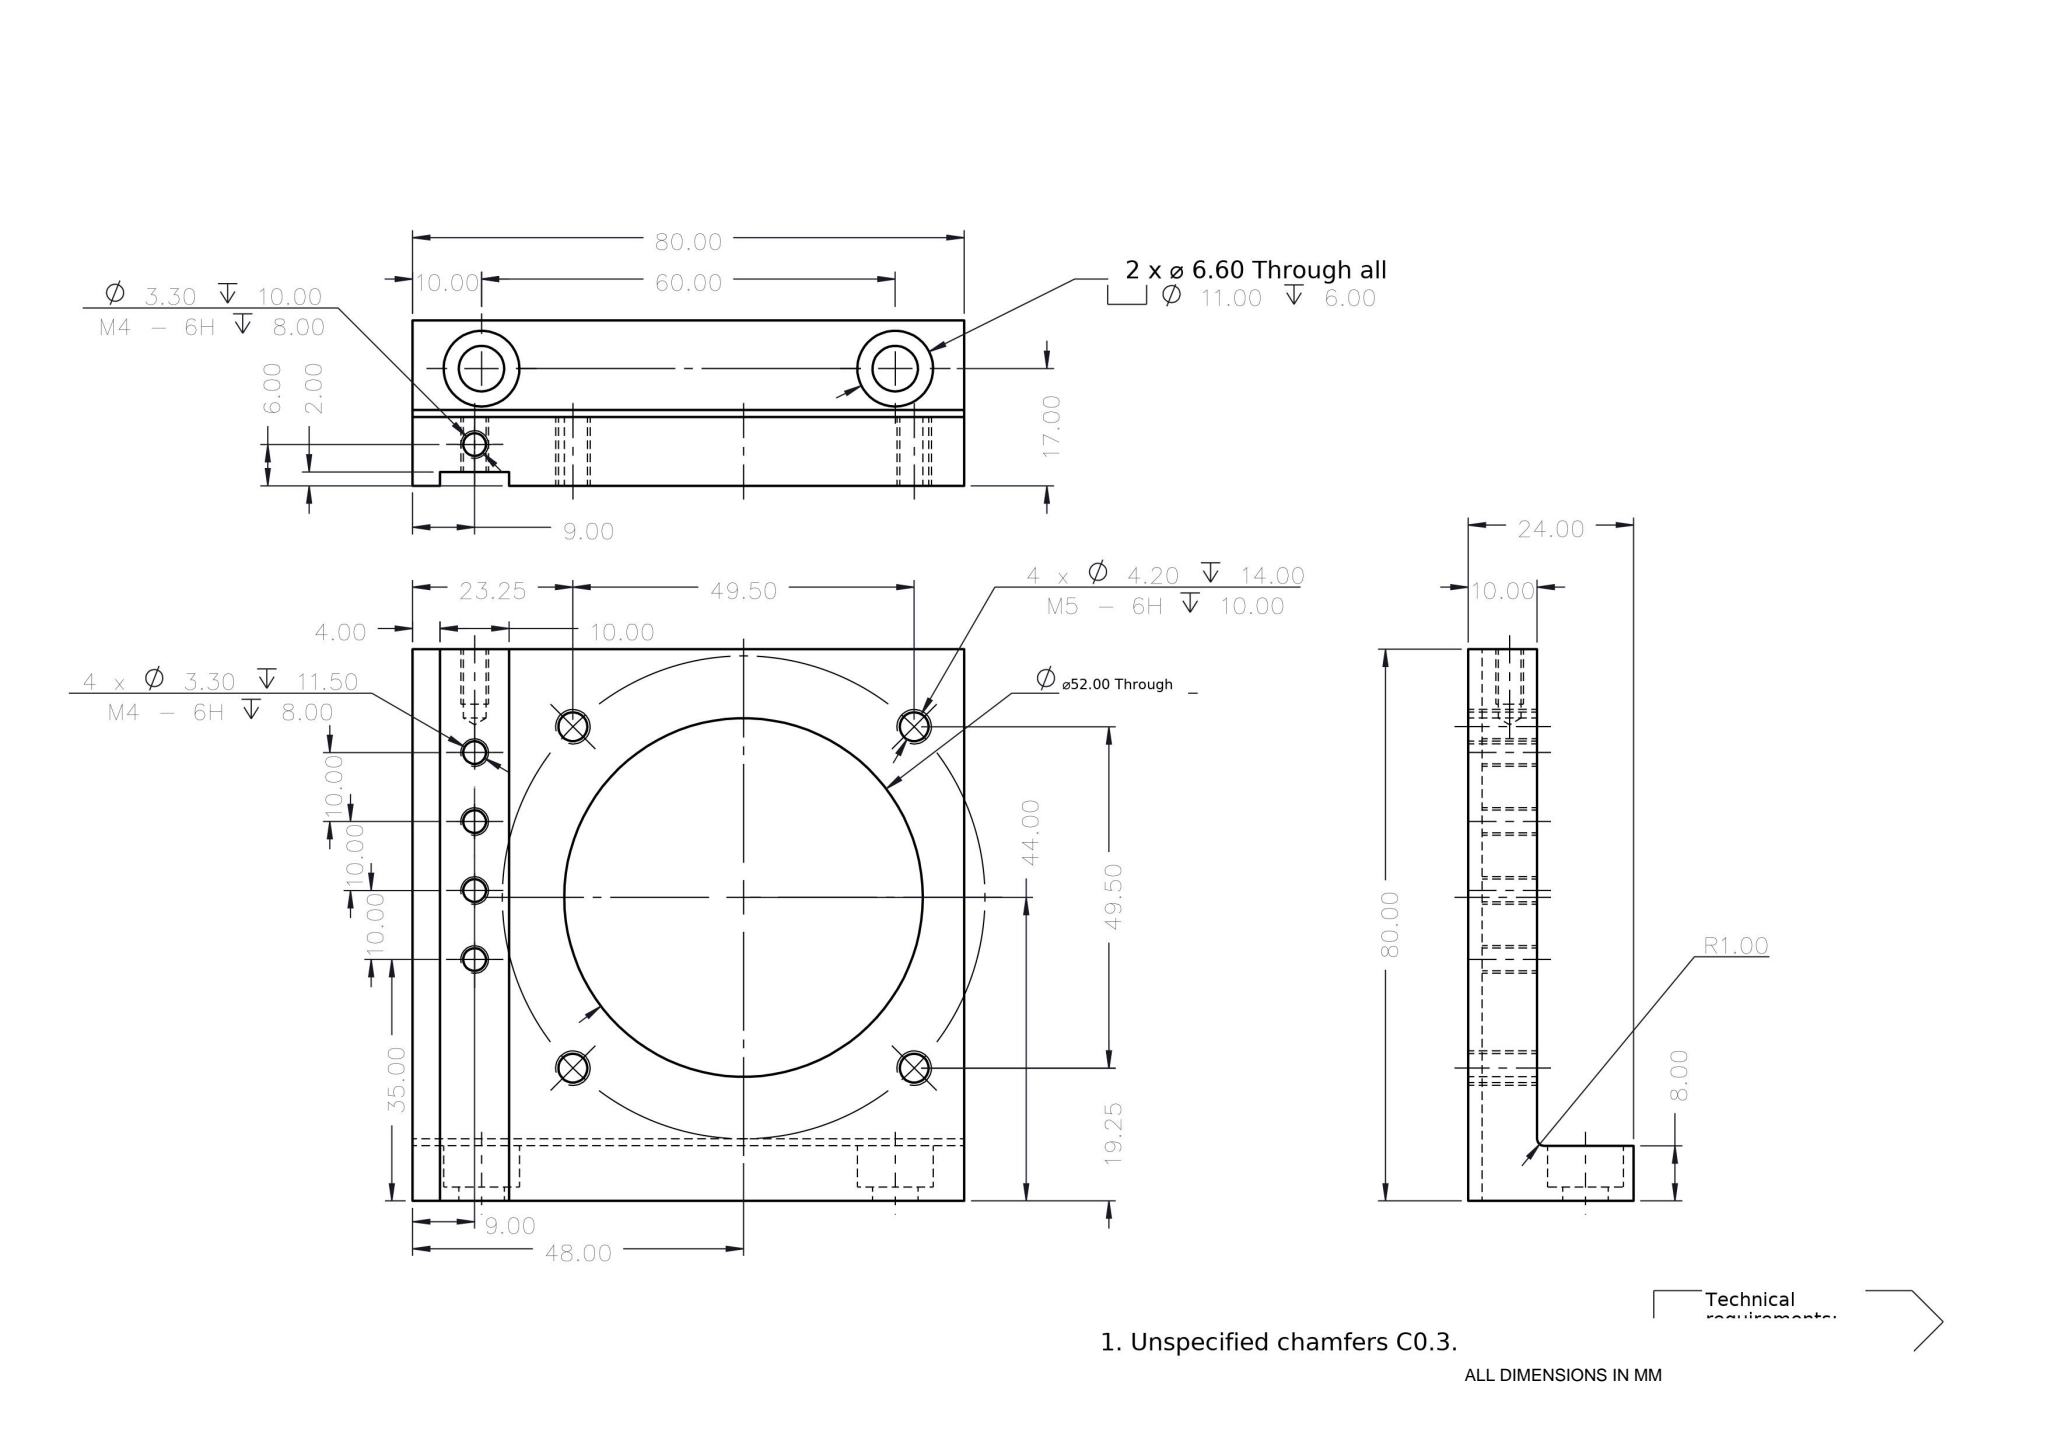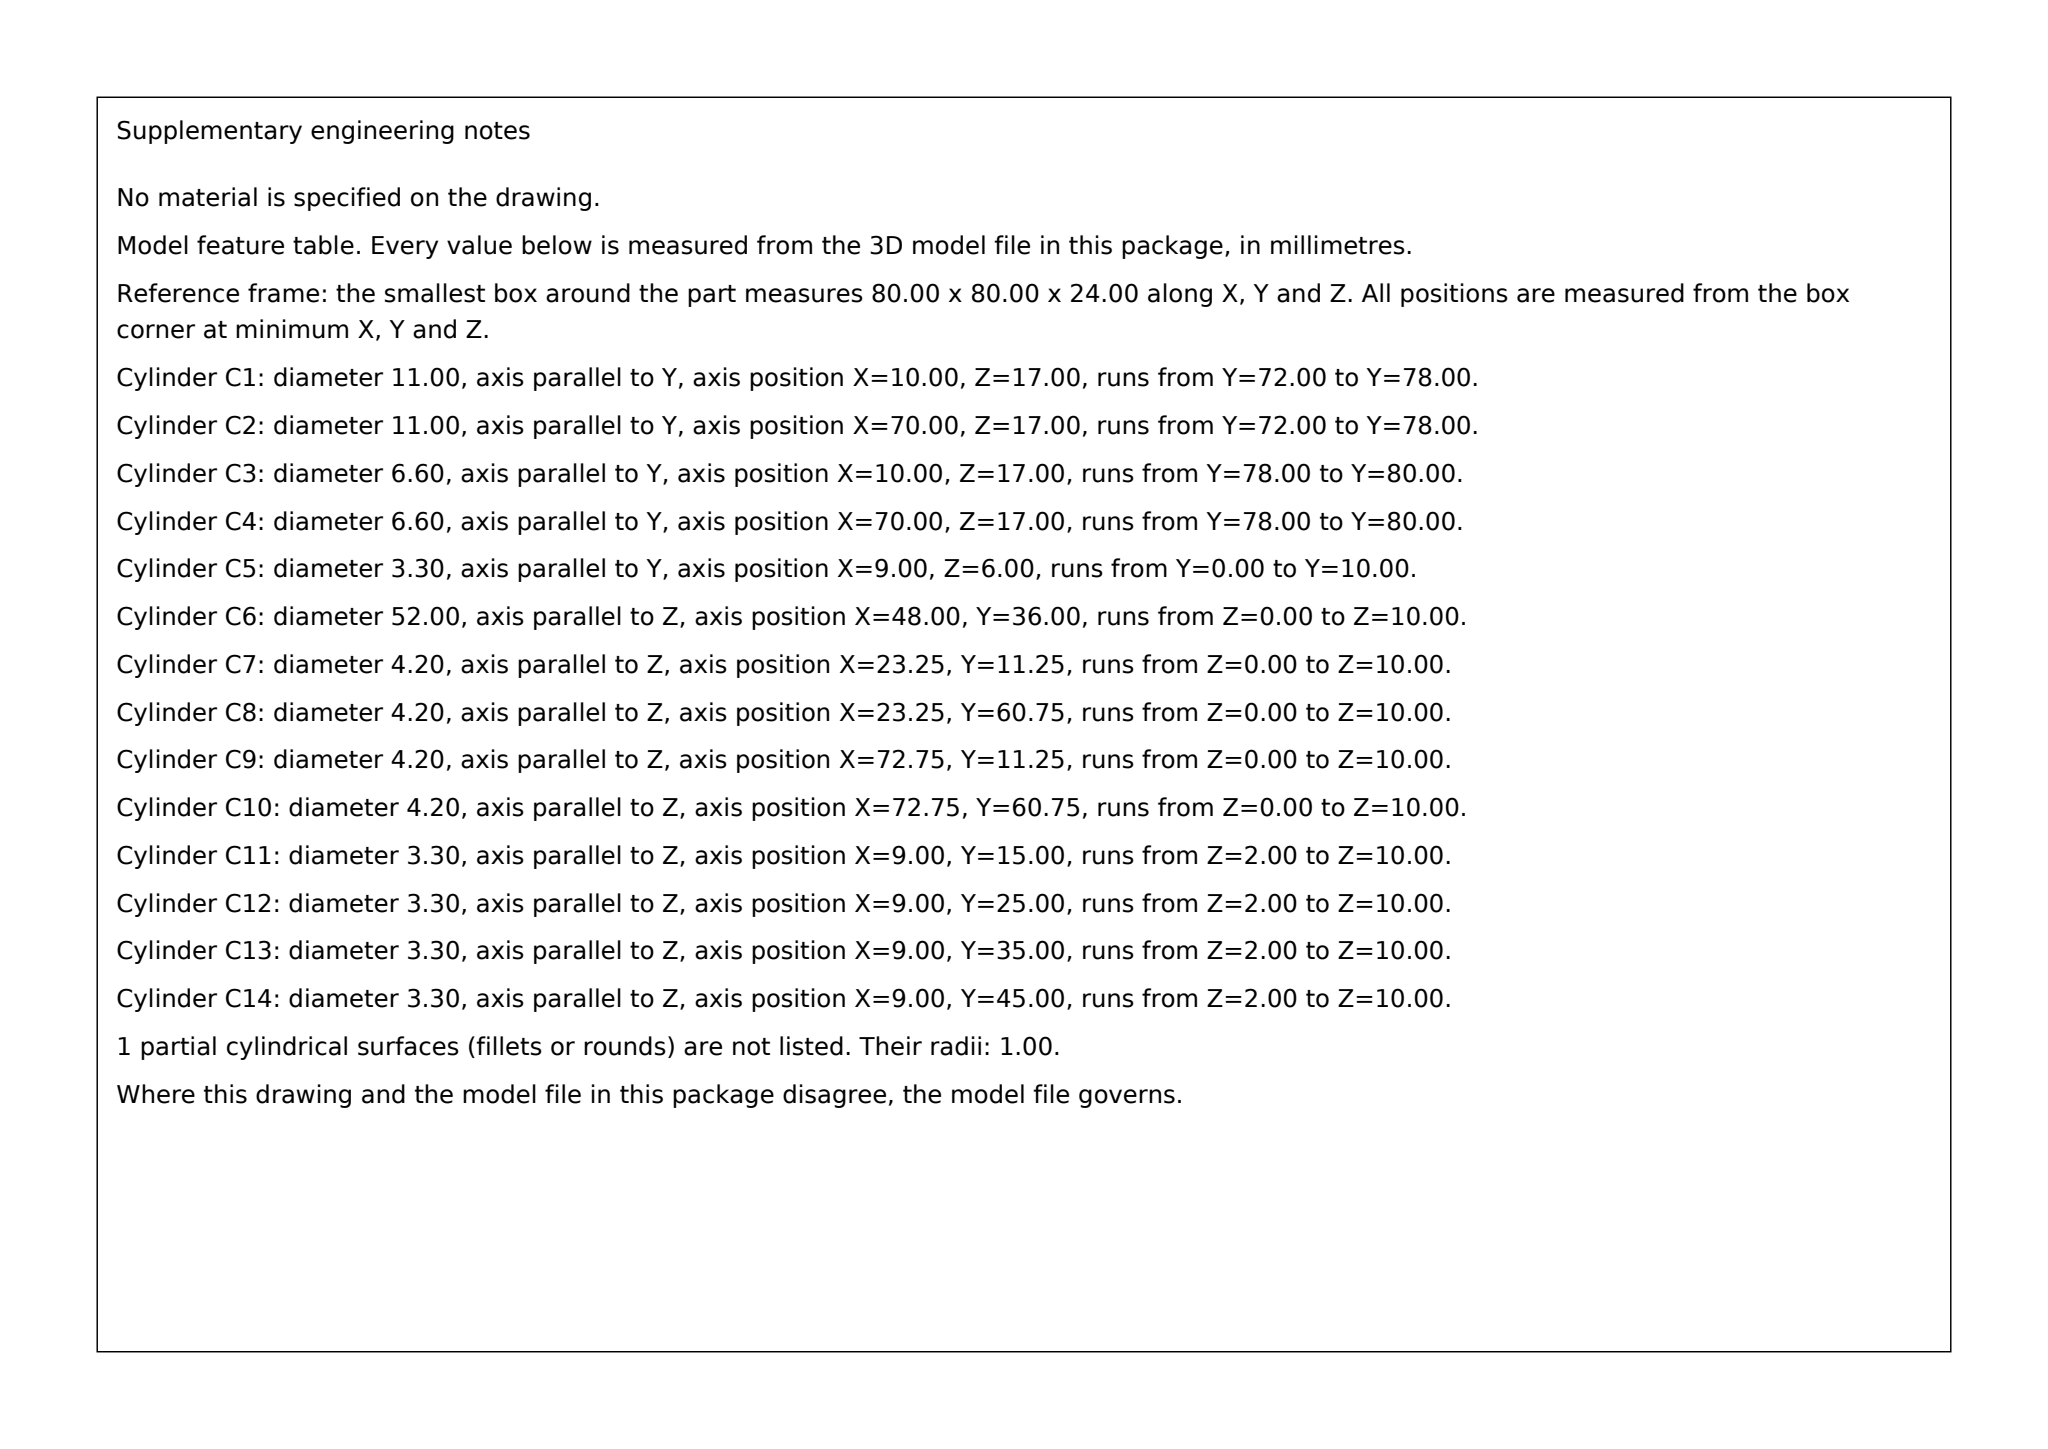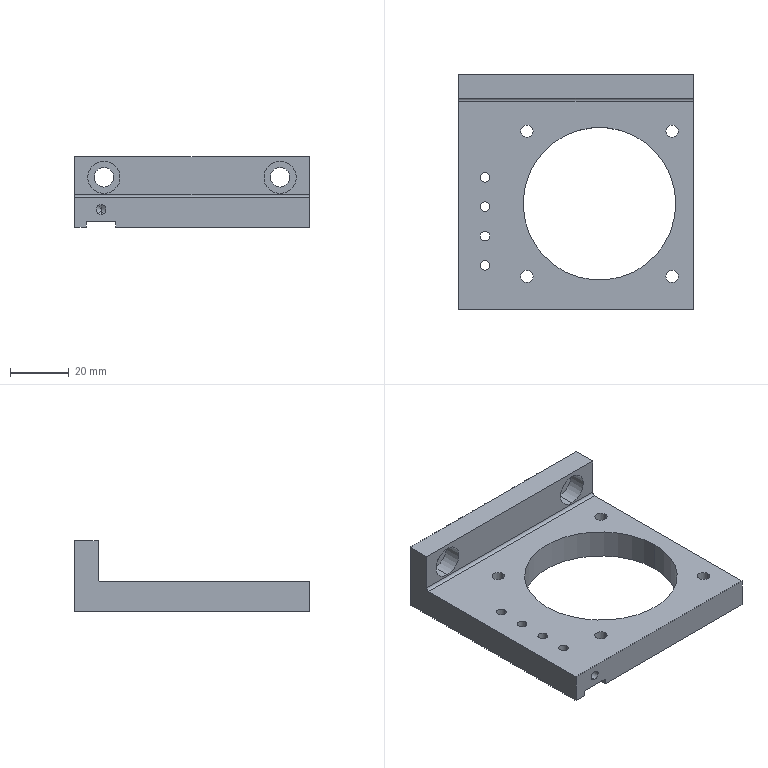Part | SolidWorks | mm | 1 solid | 45 faces | box 80 x 80 x 24 mm | volume 47947 mm3 | cylinder 29 | plane 14 | cone 2 | commonest cylinder face diameters 3.3 x10 4.2 x8 11 x4 6.6 x4 52 x2 2 x1